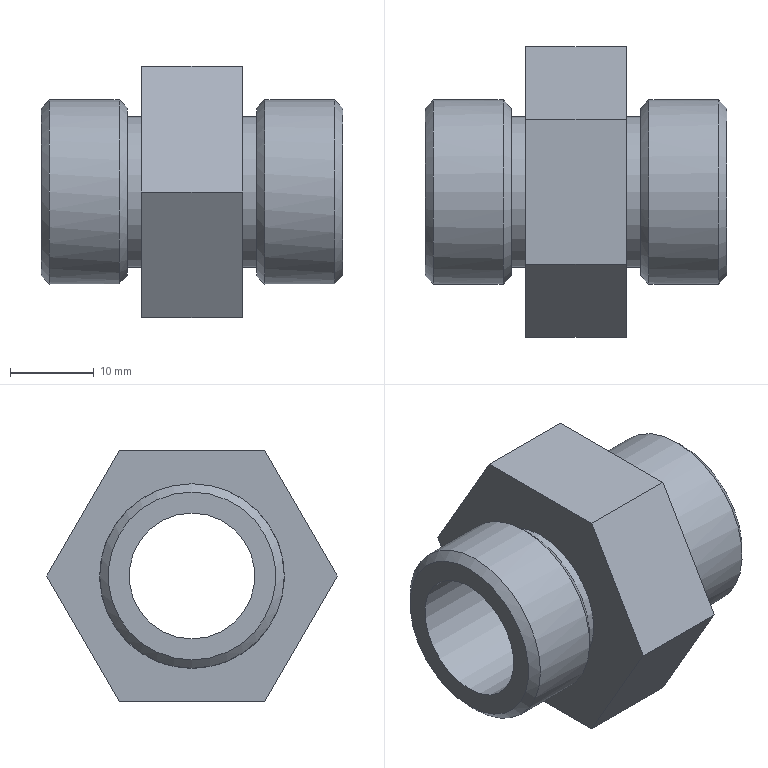Component | NX | CH3404_8-6 | 1 solid | 21 faces | volume 11553 mm3 | plane 12 | cylinder 5 | cone 4 | commonest cylinder face diameters 22 x2 18 x2 15 x1